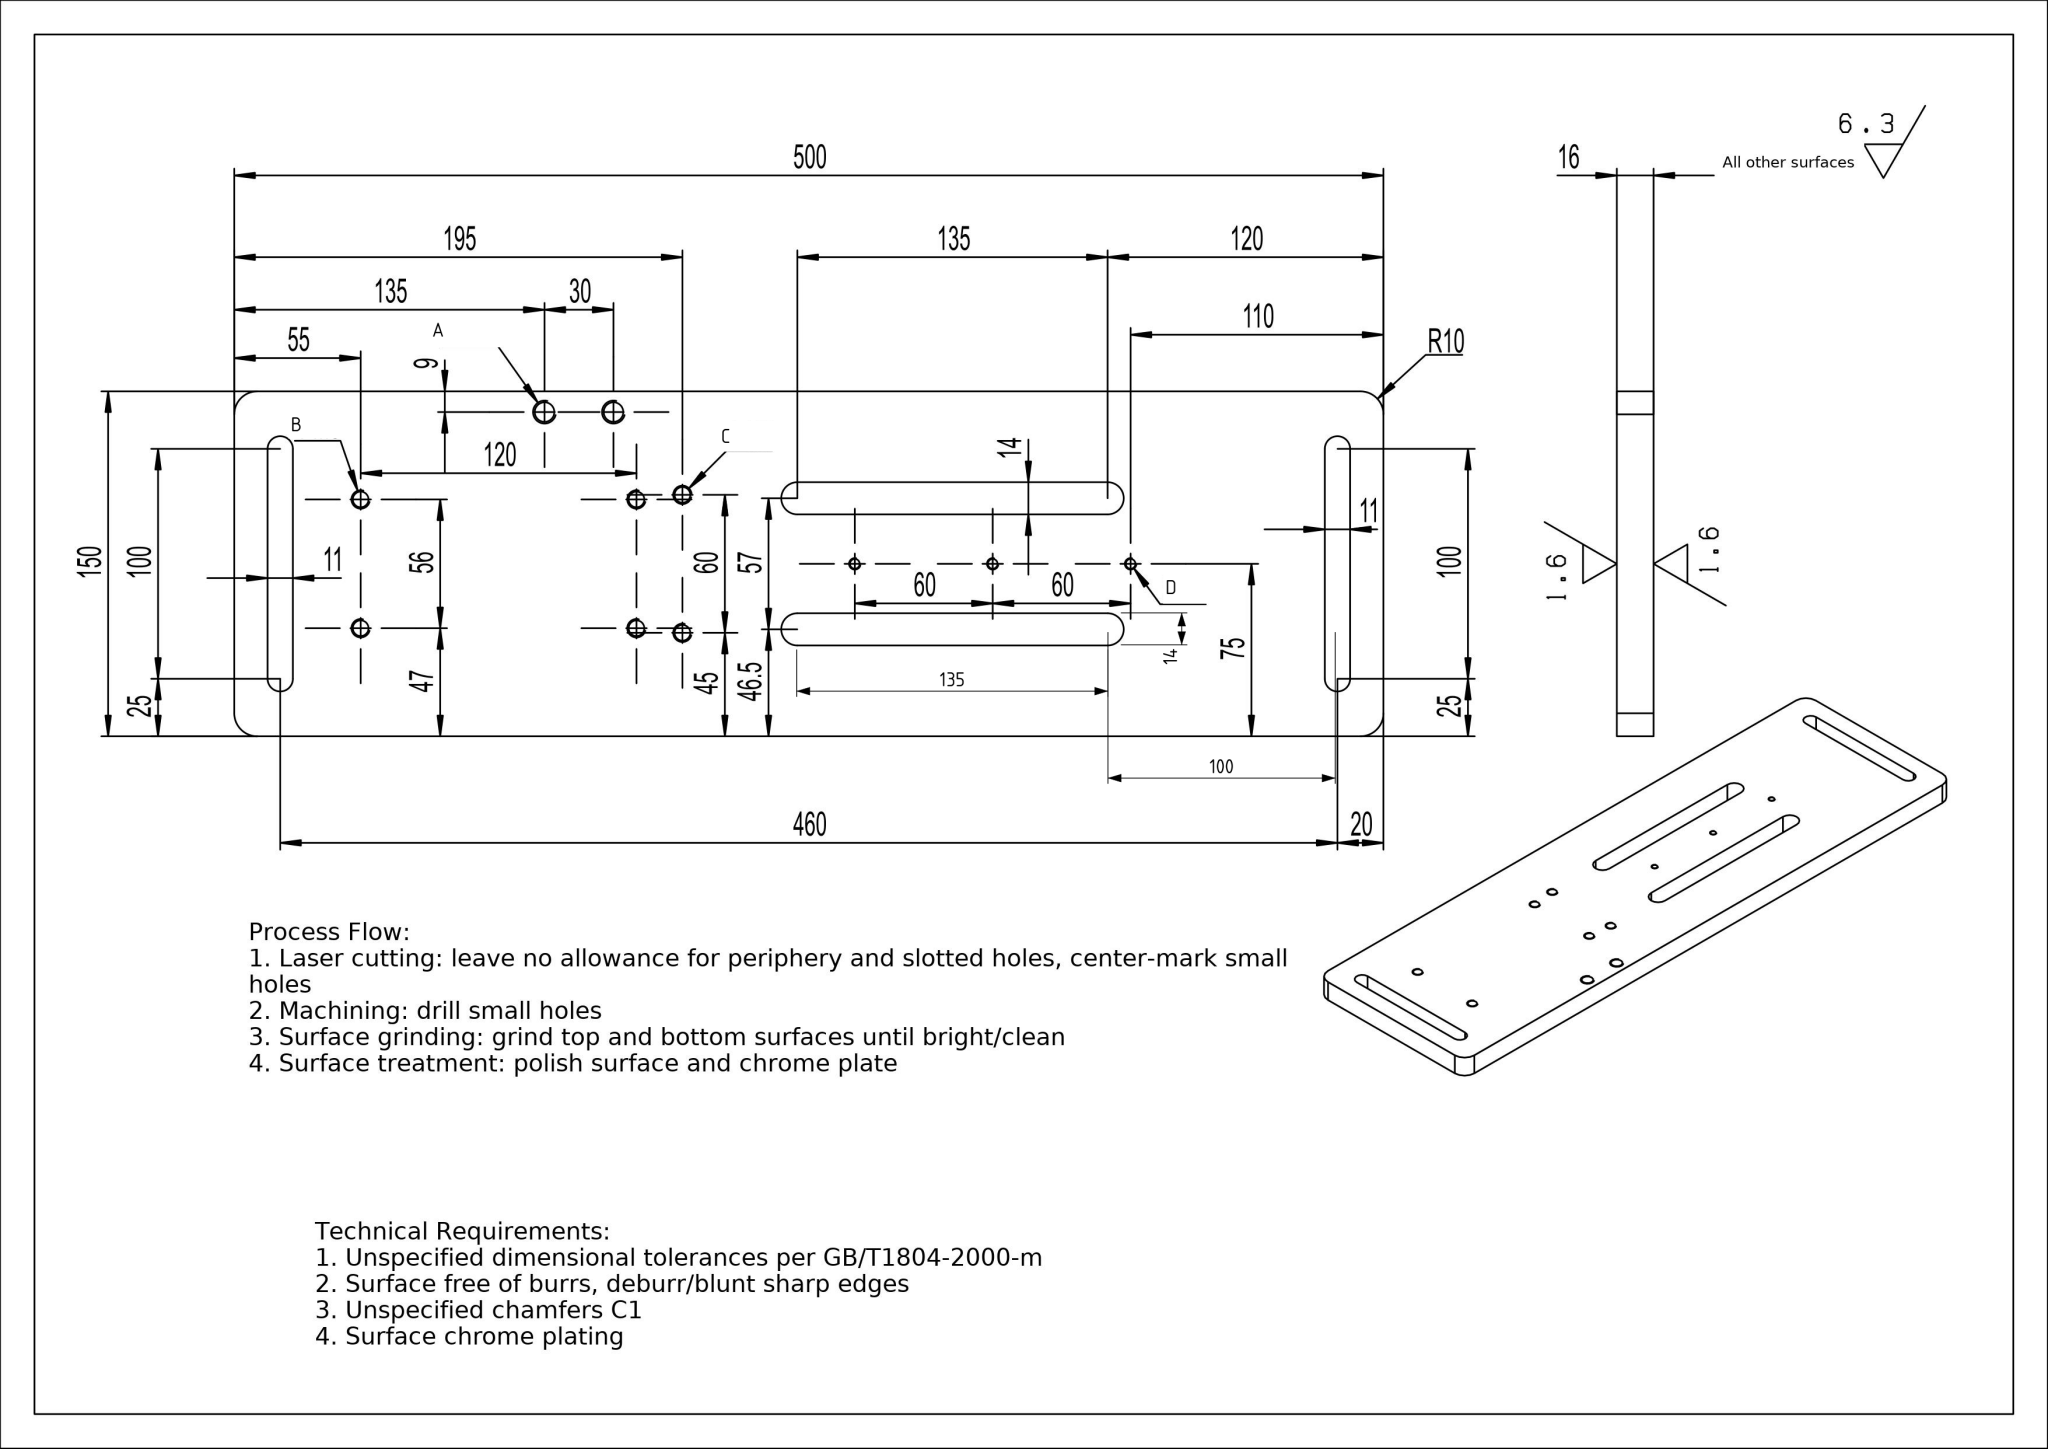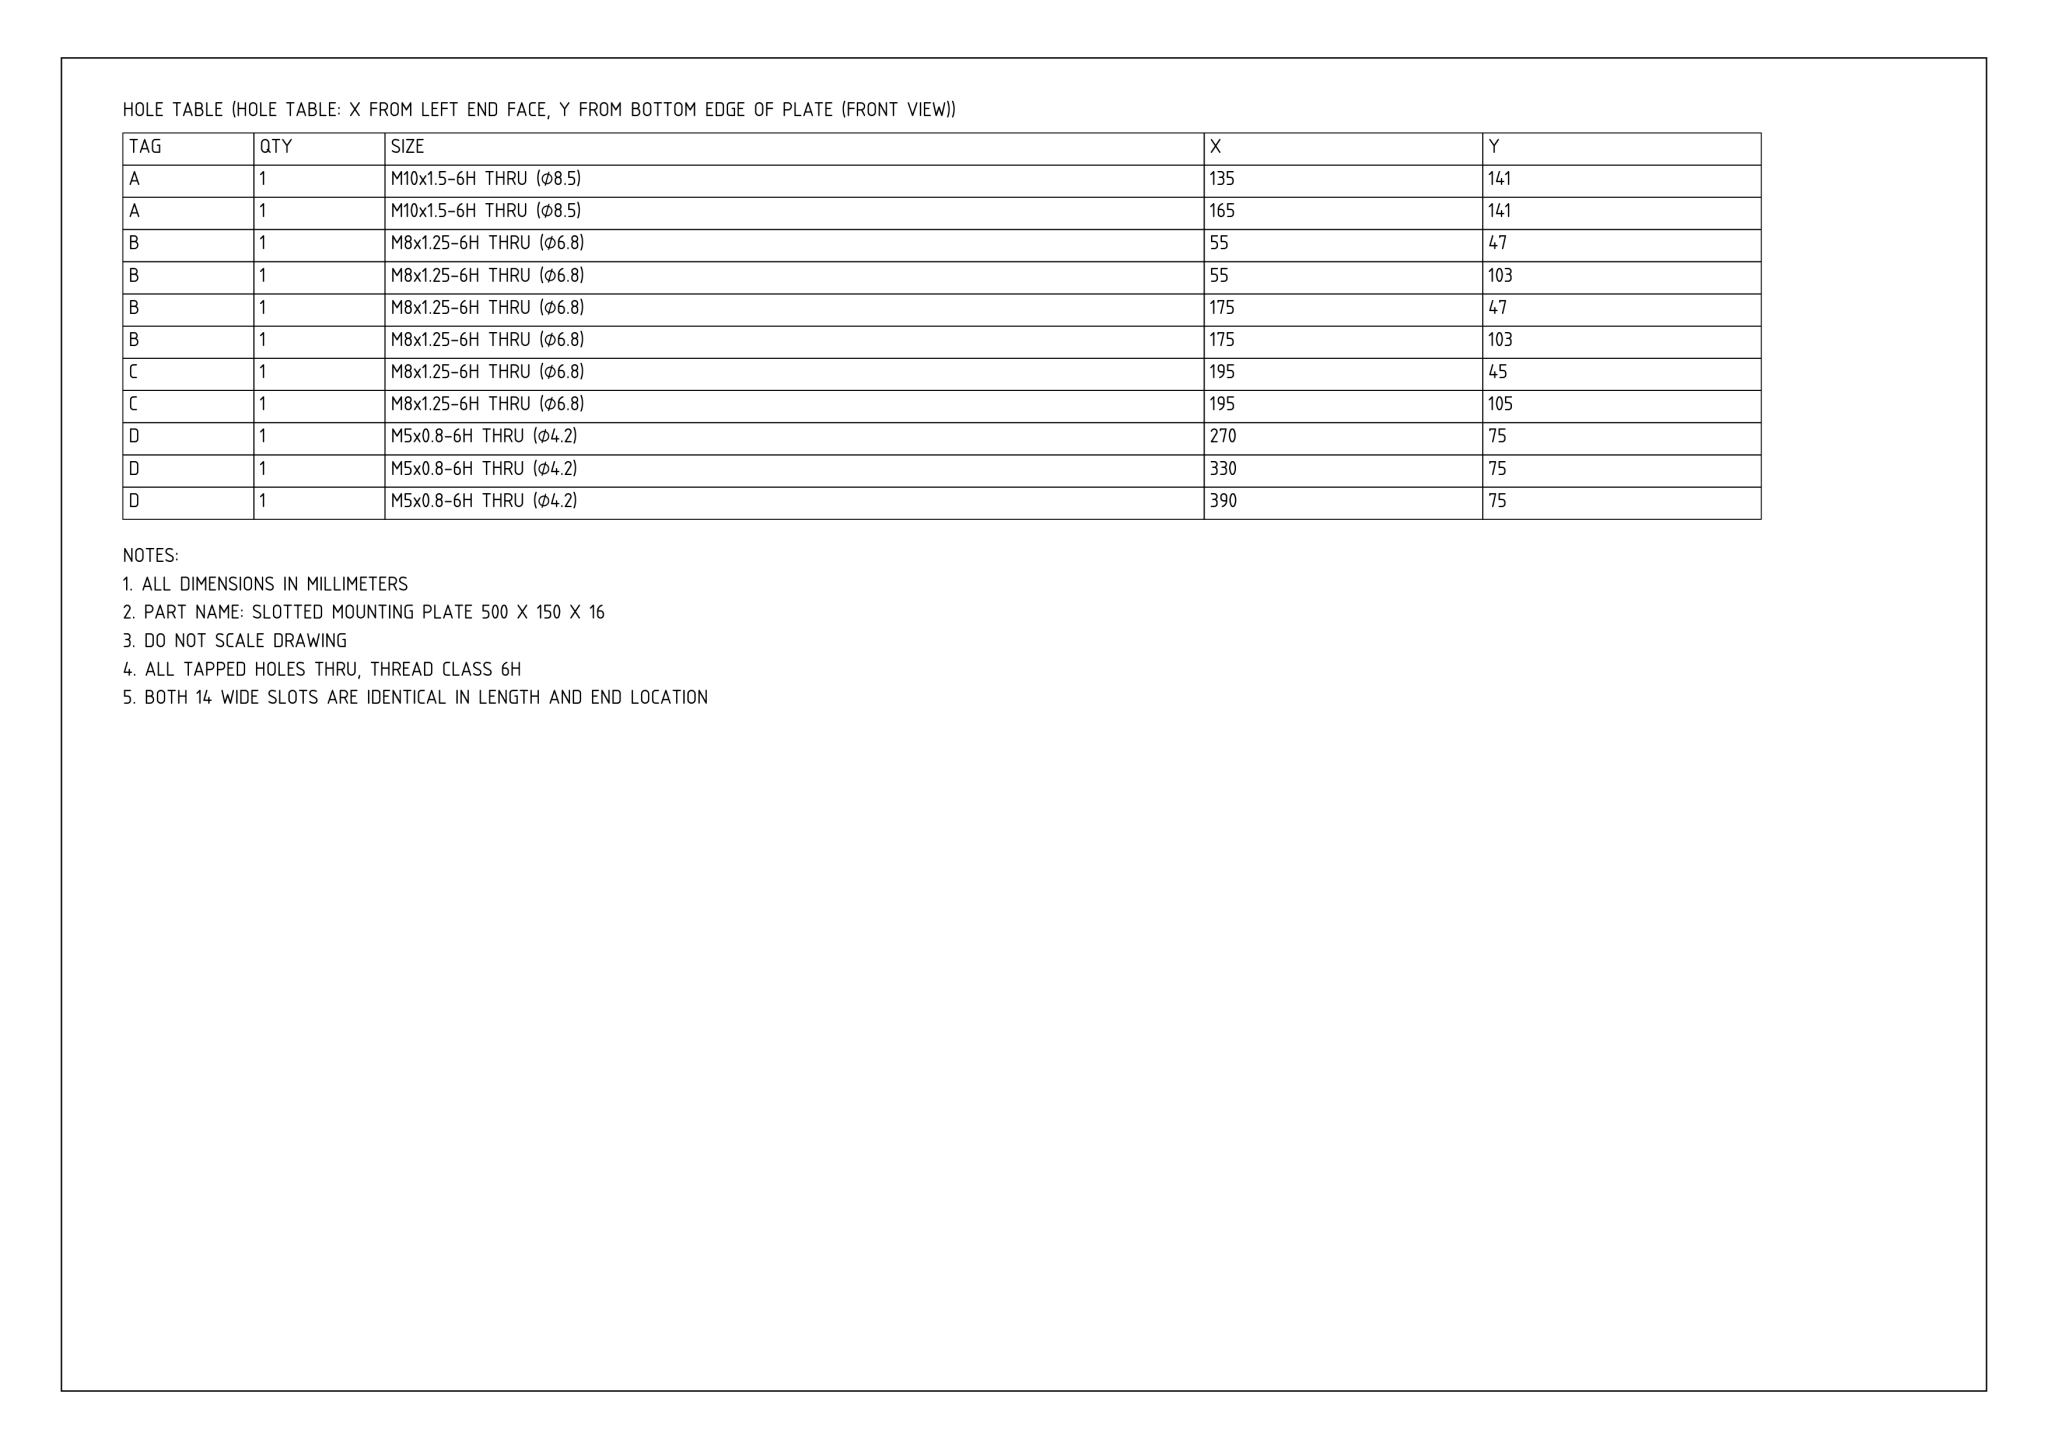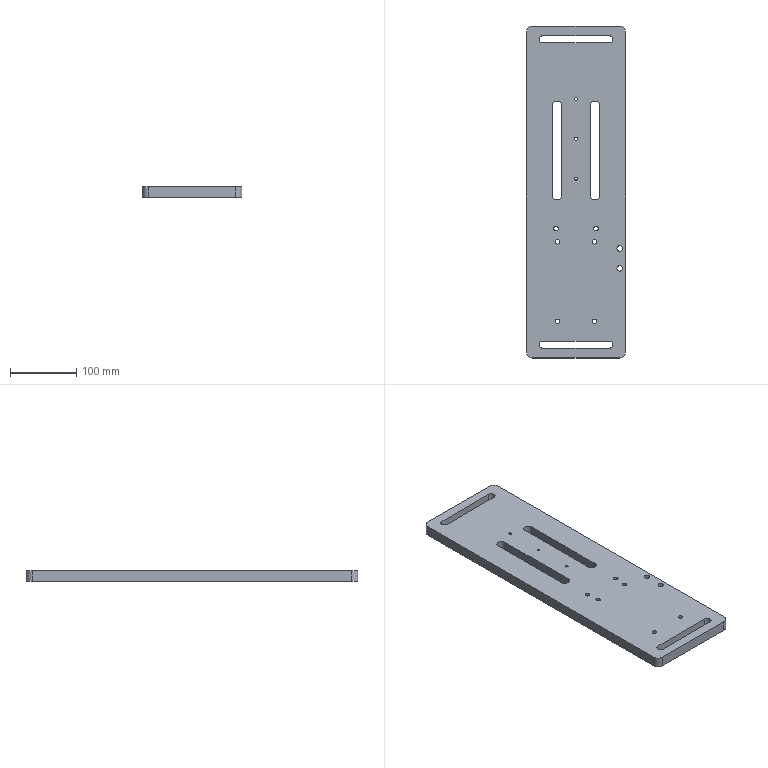Part | NX | mm | 1 solid | 37 faces | box 150 x 500 x 16 mm | volume 1089012 mm3 | cylinder 23 | plane 14 | commonest cylinder face diameters 6.8 x6 14 x4 20 x4 11 x4 4.2 x3 8.5 x2